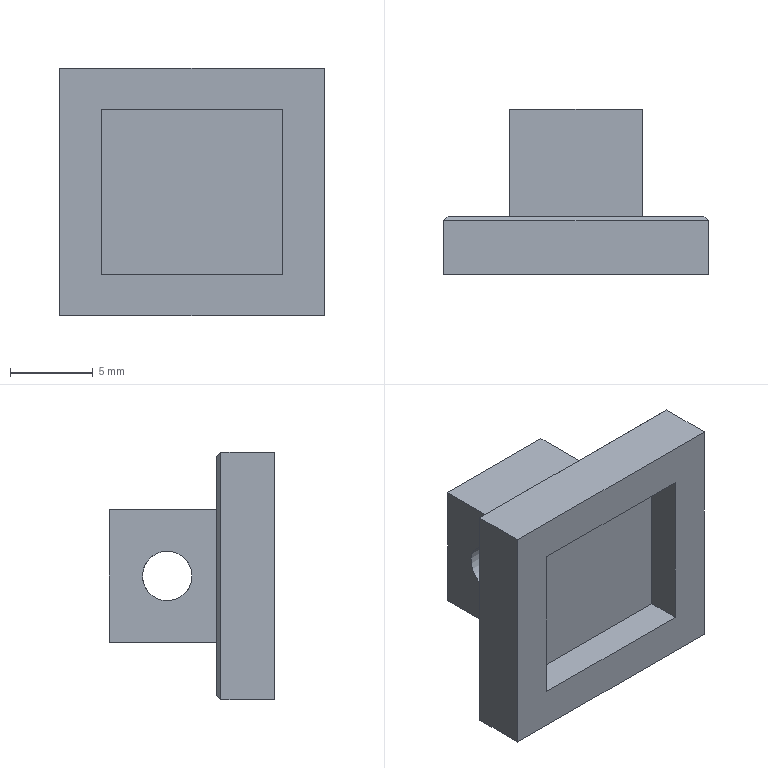Component | NX | OUTER_PISTON_BLOCK_2 | 1 solid | 21 faces | volume 978 mm3 | plane 20 | cylinder 1 | commonest cylinder face diameters 3 x1